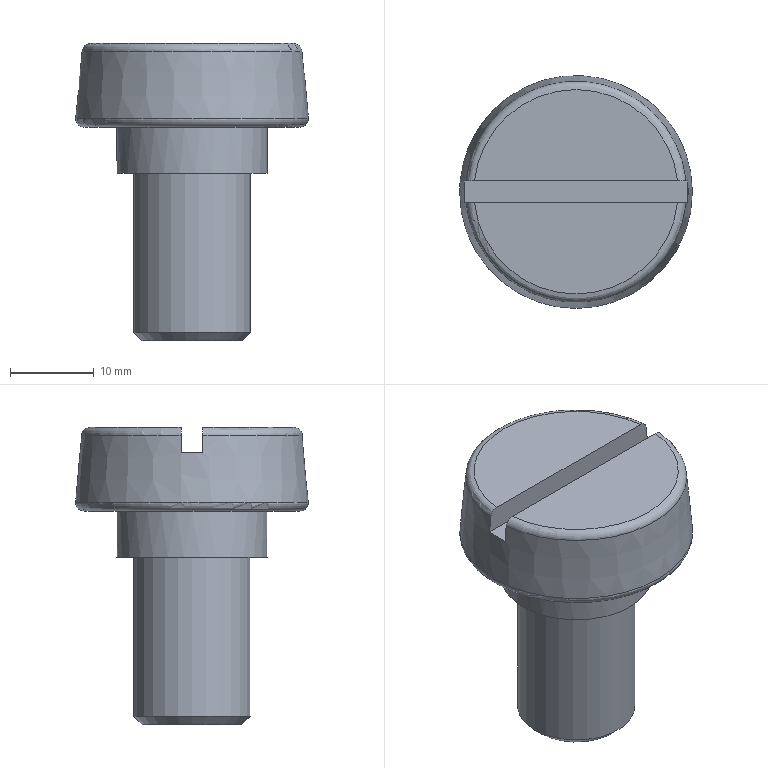Component | NX | DRILL_BUSHING_SCREW_2 | 1 solid | 15 faces | volume 9996 mm3 | plane 8 | torus 3 | cylinder 2 | cone 2 | commonest cylinder face diameters 14 x1 18 x1